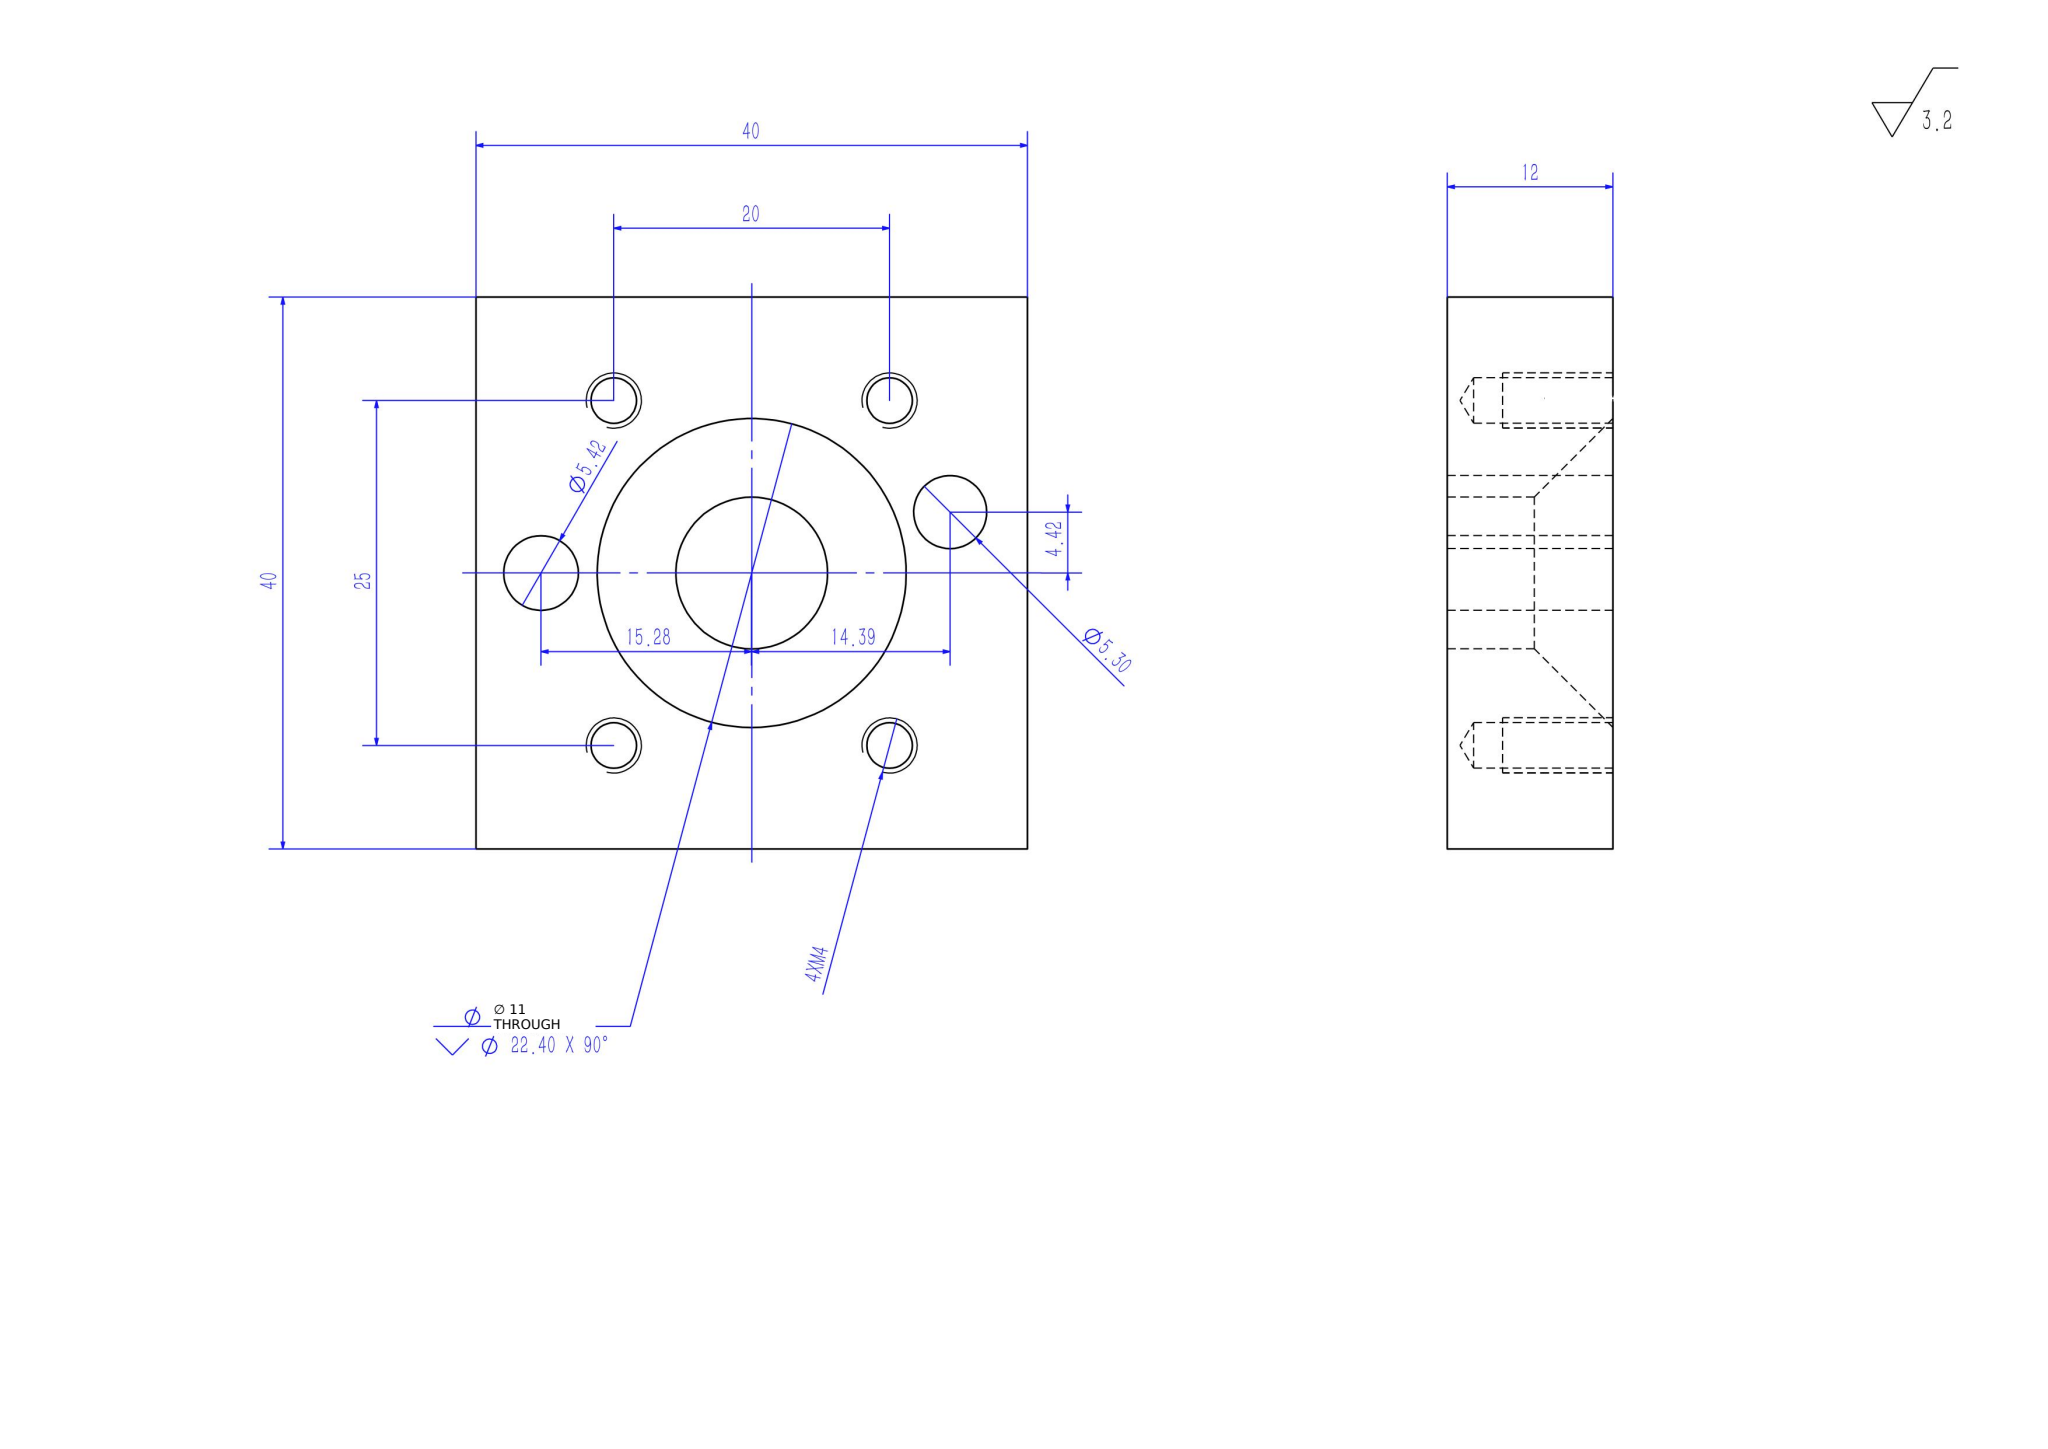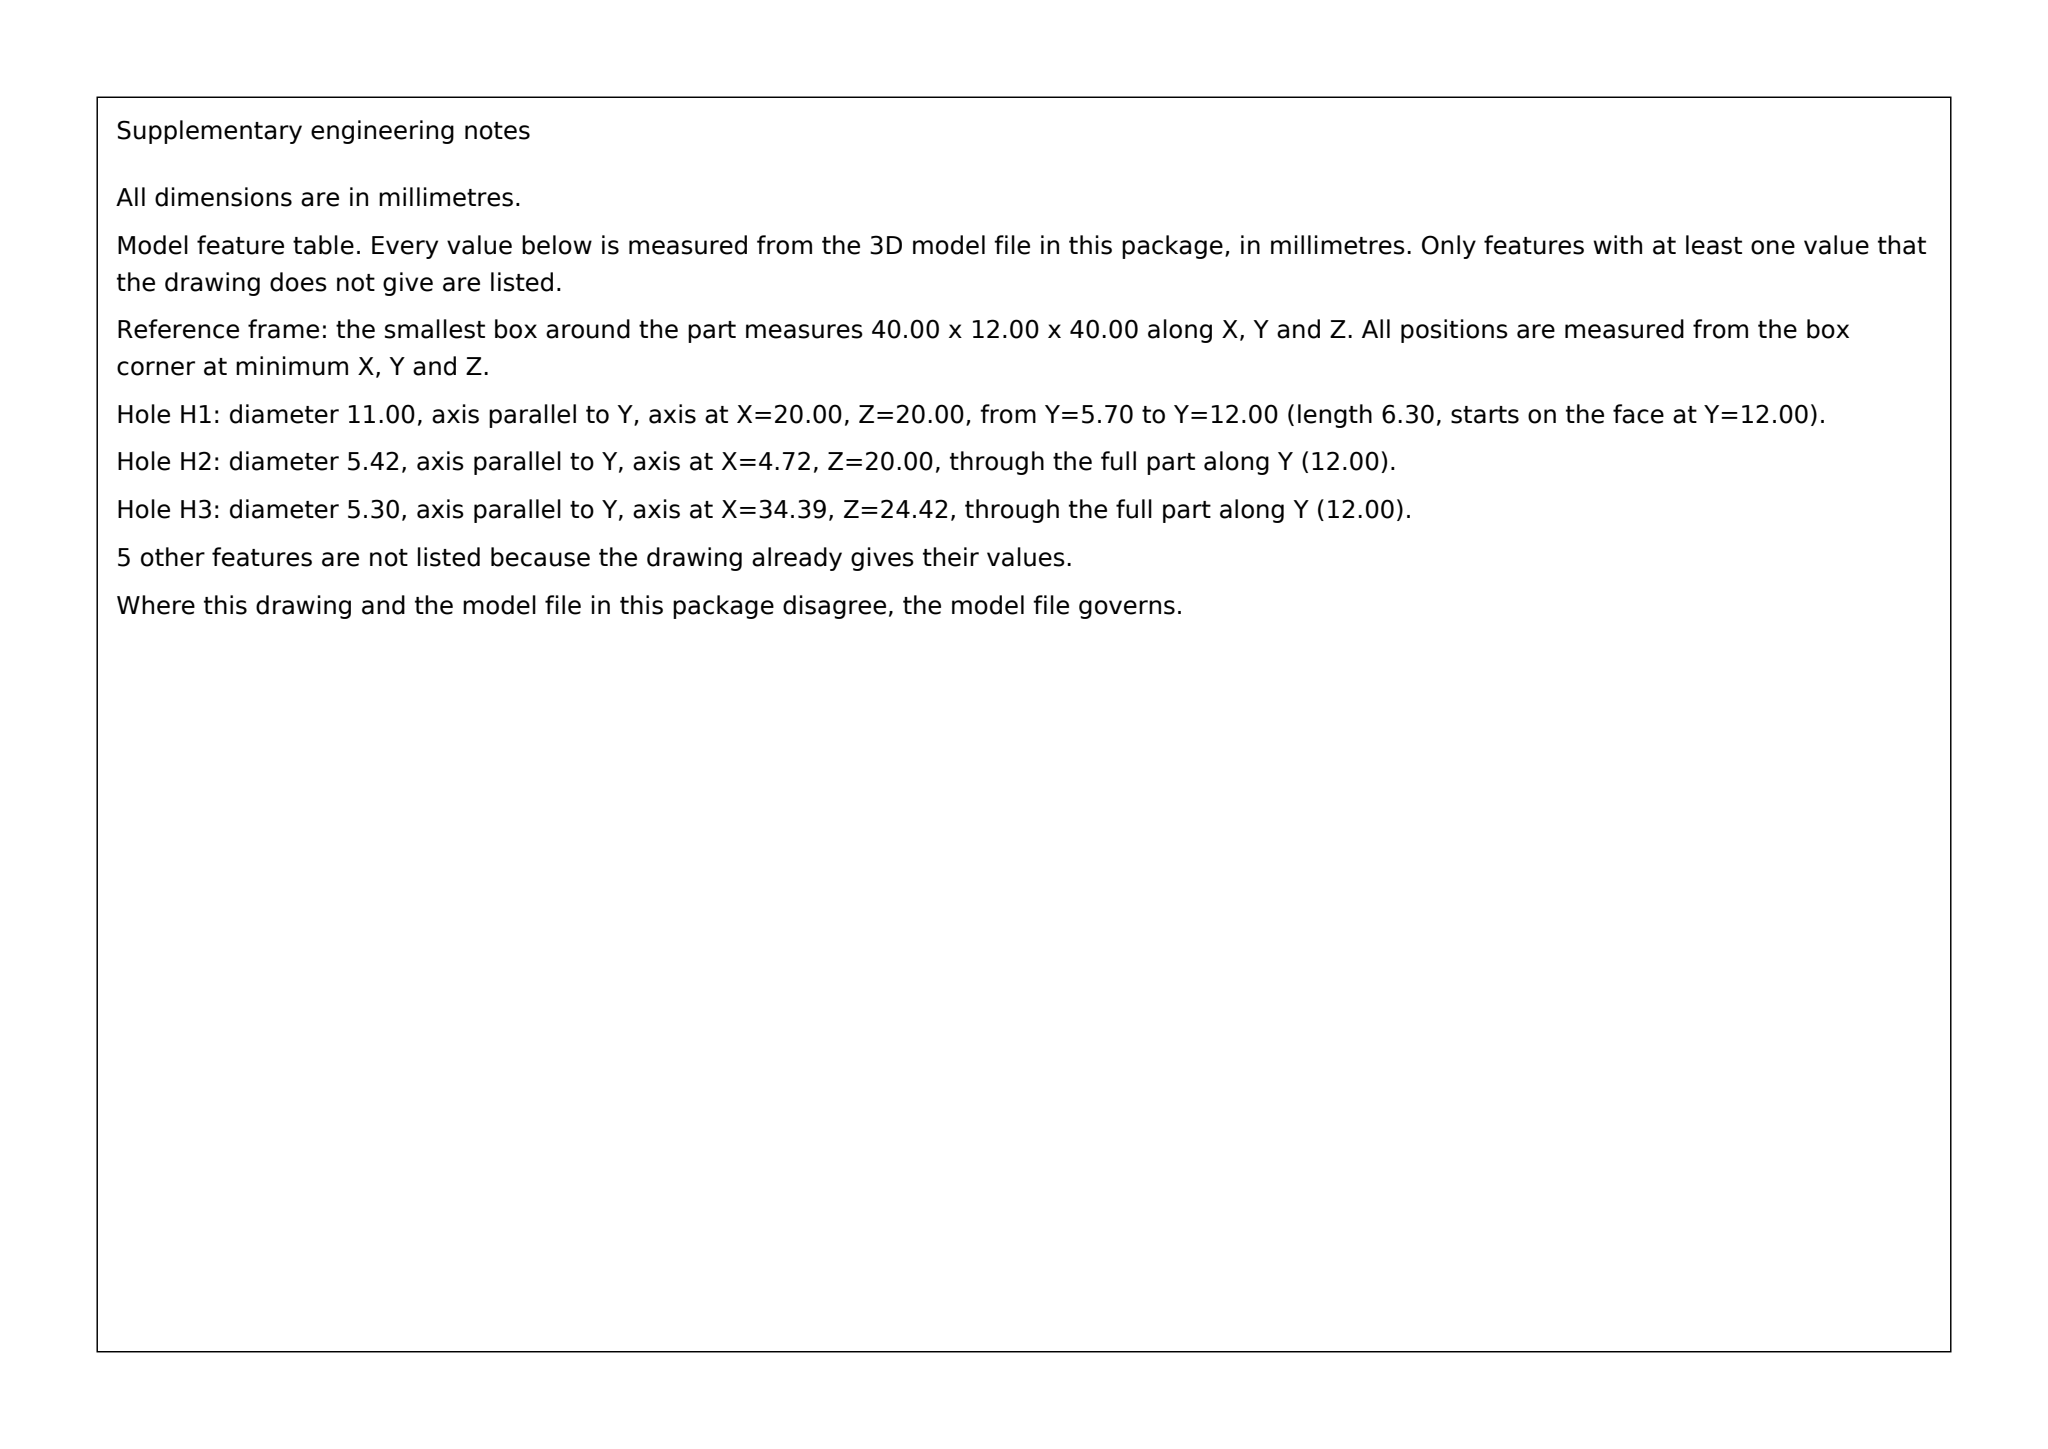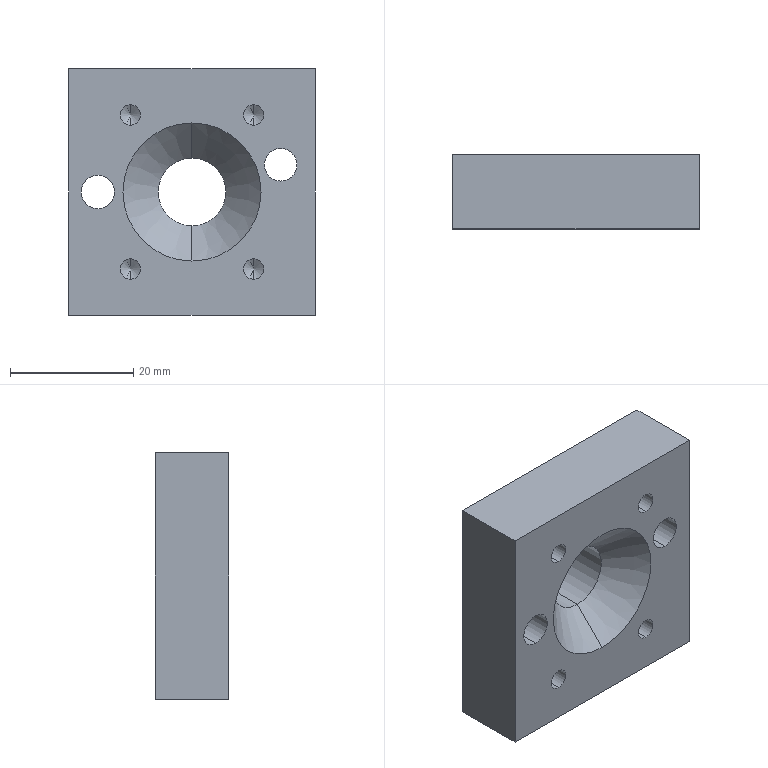Part | SolidWorks | mm | 1 solid | 30 faces | box 40 x 12 x 40 mm | volume 16406 mm3 | cylinder 14 | cone 10 | plane 6 | commonest cylinder face diameters 3.3 x8 5.298 x2 5.416 x2 11 x2
build123d program:
from build123d import *

# Parameters (mm, degrees)
SKETCH1_W                                        = 40
SKETCH1_H                                        = 40
BOSS_EXTRUDE1_DEPTH                              = 12
M10_HEX_SOCKET_HEAD_CAP_SCREW_CBORE1_D           = 11
M10_HEX_SOCKET_HEAD_CAP_SCREW_CBORE1_CSINK_D     = 22.4
M10_HEX_SOCKET_HEAD_CAP_SCREW_CBORE1_CSINK_ANGLE = 90
M4_TAPPED_HOLE1_D                                = 3.3
M4_TAPPED_HOLE1_DEPTH                            = 10.1
M4_TAPPED_HOLE1_TIP                              = 0.9914
SKETCH6_R                                        = 2.649
SKETCH6_R_2                                      = 2.708
CUT_EXTRUDE1_DEPTH                               = 80


with BuildPart() as part:
    # Sketch1 → Boss-Extrude1 (new body)
    with BuildSketch(Plane(origin=(0, 0, 0), x_dir=(1, 0, 0), z_dir=(0, 1, 0))):
        Rectangle(SKETCH1_W, SKETCH1_H)
    extrude(amount=BOSS_EXTRUDE1_DEPTH)

    # M10 Hex Socket Head Cap Screw CBORE1 (through all)
    with Locations(Plane(origin=(0, 0, 0), x_dir=(-1, 0, 0), z_dir=(0, -1, 0))):
        with Locations((0, 0)):
            CounterSinkHole(M10_HEX_SOCKET_HEAD_CAP_SCREW_CBORE1_D / 2, M10_HEX_SOCKET_HEAD_CAP_SCREW_CBORE1_CSINK_D / 2, counter_sink_angle=M10_HEX_SOCKET_HEAD_CAP_SCREW_CBORE1_CSINK_ANGLE)

    # M4 Tapped Hole1
    with Locations(Plane(origin=(0, 0, 0), x_dir=(-1, 0, 0), z_dir=(0, -1, 0))):
        with Locations((-10, 12.5), (10, 12.5), (-10, -12.5), (10, -12.5)):
            Hole(M4_TAPPED_HOLE1_D / 2, depth=M4_TAPPED_HOLE1_DEPTH)
            with Locations((0, 0, -(M4_TAPPED_HOLE1_DEPTH + M4_TAPPED_HOLE1_TIP / 2))):  # 118° drill point
                Cone(0, M4_TAPPED_HOLE1_D / 2, M4_TAPPED_HOLE1_TIP, mode=Mode.SUBTRACT)

    # Sketch6 → Cut-Extrude1 (cut)
    with BuildSketch(Plane(origin=(0, 0, 0), x_dir=(-1, 0, 0), z_dir=(0, -1, 0))):
        with Locations(Location((-14.39, -4.415, 0), (0, 0, 90))):
            Circle(SKETCH6_R)
        with Locations(Location((15.279, 0, 0), (0, 0, 90))):
            Circle(SKETCH6_R_2)
    extrude(amount=-CUT_EXTRUDE1_DEPTH, mode=Mode.SUBTRACT)


solid = part.part
STEP:
#1=CARTESIAN_POINT('',(14.39,12.,7.064));
#2=VERTEX_POINT('',#1);
#3=CARTESIAN_POINT('',(14.39,12.,1.766));
#4=VERTEX_POINT('',#3);
#5=CARTESIAN_POINT('',(14.39,12.,4.415));
#6=DIRECTION('',(0.,-1.,0.));
#7=DIRECTION('',(0.,0.,-1.));
#8=AXIS2_PLACEMENT_3D('',#5,#6,#7);
#9=CIRCLE('',#8,2.649);
#10=EDGE_CURVE('',#2,#4,#9,.T.);
#11=ORIENTED_EDGE('',*,*,#10,.F.);
#12=CARTESIAN_POINT('',(14.39,0.,7.064));
#13=VERTEX_POINT('',#12);
#14=CARTESIAN_POINT('',(14.39,80.,7.064));
#15=DIRECTION('',(0.,-1.,0.));
#16=VECTOR('',#15,1000.);
#17=LINE('',#14,#16);
#18=EDGE_CURVE('',#2,#13,#17,.T.);
#19=ORIENTED_EDGE('',*,*,#18,.T.);
#20=CARTESIAN_POINT('',(14.39,0.,1.766));
#21=VERTEX_POINT('',#20);
#22=CARTESIAN_POINT('',(14.39,0.,4.415));
#23=DIRECTION('',(0.,-1.,0.));
#24=DIRECTION('',(0.,0.,-1.));
#25=AXIS2_PLACEMENT_3D('',#22,#23,#24);
#26=CIRCLE('',#25,2.649);
#27=EDGE_CURVE('',#13,#21,#26,.T.);
#28=ORIENTED_EDGE('',*,*,#27,.T.);
#29=CARTESIAN_POINT('',(14.39,80.,1.766));
#30=DIRECTION('',(0.,-1.,0.));
#31=VECTOR('',#30,1000.);
#32=LINE('',#29,#31);
#33=EDGE_CURVE('',#4,#21,#32,.T.);
#34=ORIENTED_EDGE('',*,*,#33,.F.);
#35=EDGE_LOOP('',(#11,#19,#28,#34));
#36=FACE_OUTER_BOUND('',#35,.T.);
#37=CARTESIAN_POINT('',(14.39,80.,4.415));
#38=DIRECTION('',(0.,-1.,0.));
#39=DIRECTION('',(0.,0.,-1.));
#40=AXIS2_PLACEMENT_3D('',#37,#38,#39);
#41=CYLINDRICAL_SURFACE('',#40,2.649);
#42=ADVANCED_FACE('',(#36),#41,.F.);
#43=CARTESIAN_POINT('',(-15.279,12.,2.708));
#44=VERTEX_POINT('',#43);
#45=CARTESIAN_POINT('',(-15.279,12.,-2.708));
#46=VERTEX_POINT('',#45);
#47=CARTESIAN_POINT('',(-15.279,12.,0.));
#48=DIRECTION('',(0.,-1.,0.));
#49=DIRECTION('',(0.,0.,-1.));
#50=AXIS2_PLACEMENT_3D('',#47,#48,#49);
#51=CIRCLE('',#50,2.708);
#52=EDGE_CURVE('',#44,#46,#51,.T.);
#53=ORIENTED_EDGE('',*,*,#52,.F.);
#54=CARTESIAN_POINT('',(-15.279,0.,2.708));
#55=VERTEX_POINT('',#54);
#56=CARTESIAN_POINT('',(-15.279,80.,2.708));
#57=DIRECTION('',(0.,-1.,0.));
#58=VECTOR('',#57,1000.);
#59=LINE('',#56,#58);
#60=EDGE_CURVE('',#44,#55,#59,.T.);
#61=ORIENTED_EDGE('',*,*,#60,.T.);
#62=CARTESIAN_POINT('',(-15.279,0.,-2.708));
#63=VERTEX_POINT('',#62);
#64=CARTESIAN_POINT('',(-15.279,0.,0.));
#65=DIRECTION('',(0.,-1.,0.));
#66=DIRECTION('',(0.,0.,-1.));
#67=AXIS2_PLACEMENT_3D('',#64,#65,#66);
#68=CIRCLE('',#67,2.708);
#69=EDGE_CURVE('',#55,#63,#68,.T.);
#70=ORIENTED_EDGE('',*,*,#69,.T.);
#71=CARTESIAN_POINT('',(-15.279,80.,-2.708));
#72=DIRECTION('',(0.,-1.,0.));
#73=VECTOR('',#72,1000.);
#74=LINE('',#71,#73);
#75=EDGE_CURVE('',#46,#63,#74,.T.);
#76=ORIENTED_EDGE('',*,*,#75,.F.);
#77=EDGE_LOOP('',(#53,#61,#70,#76));
#78=FACE_OUTER_BOUND('',#77,.T.);
#79=CARTESIAN_POINT('',(-15.279,80.,0.));
#80=DIRECTION('',(0.,-1.,0.));
#81=DIRECTION('',(0.,0.,-1.));
#82=AXIS2_PLACEMENT_3D('',#79,#80,#81);
#83=CYLINDRICAL_SURFACE('',#82,2.708);
#84=ADVANCED_FACE('',(#78),#83,.F.);
#85=CARTESIAN_POINT('',(10.,10.1,-10.85));
#86=VERTEX_POINT('',#85);
#87=CARTESIAN_POINT('',(10.,10.1,-14.15));
#88=VERTEX_POINT('',#87);
#89=CARTESIAN_POINT('',(10.,10.1,-12.5));
#90=DIRECTION('',(0.,-1.,0.));
#91=DIRECTION('',(0.,0.,-1.));
#92=AXIS2_PLACEMENT_3D('',#89,#90,#91);
#93=CIRCLE('',#92,1.65);
#94=EDGE_CURVE('',#86,#88,#93,.T.);
#95=ORIENTED_EDGE('',*,*,#94,.F.);
#96=CARTESIAN_POINT('',(10.,-0.,-10.85));
#97=VERTEX_POINT('',#96);
#98=CARTESIAN_POINT('',(10.,0.,-10.85));
#99=DIRECTION('',(0.,-1.,0.));
#100=VECTOR('',#99,1000.);
#101=LINE('',#98,#100);
#102=EDGE_CURVE('',#86,#97,#101,.T.);
#103=ORIENTED_EDGE('',*,*,#102,.T.);
#104=CARTESIAN_POINT('',(10.,-0.,-14.15));
#105=VERTEX_POINT('',#104);
#106=CARTESIAN_POINT('',(10.,-0.,-12.5));
#107=DIRECTION('',(0.,-1.,0.));
#108=DIRECTION('',(0.,0.,-1.));
#109=AXIS2_PLACEMENT_3D('',#106,#107,#108);
#110=CIRCLE('',#109,1.65);
#111=EDGE_CURVE('',#97,#105,#110,.T.);
#112=ORIENTED_EDGE('',*,*,#111,.T.);
#113=CARTESIAN_POINT('',(10.,0.,-14.15));
#114=DIRECTION('',(0.,-1.,0.));
#115=VECTOR('',#114,1000.);
#116=LINE('',#113,#115);
#117=EDGE_CURVE('',#88,#105,#116,.T.);
#118=ORIENTED_EDGE('',*,*,#117,.F.);
#119=EDGE_LOOP('',(#95,#103,#112,#118));
#120=FACE_OUTER_BOUND('',#119,.T.);
#121=CARTESIAN_POINT('',(10.,0.,-12.5));
#122=DIRECTION('',(0.,-1.,0.));
#123=DIRECTION('',(0.,0.,-1.));
#124=AXIS2_PLACEMENT_3D('',#121,#122,#123);
#125=CYLINDRICAL_SURFACE('',#124,1.65);
#126=ADVANCED_FACE('',(#120),#125,.F.);
#127=CARTESIAN_POINT('',(10.,11.091,-12.5));
#128=VERTEX_POINT('',#127);
#129=CARTESIAN_POINT('',(10.,10.1,-14.15));
#130=DIRECTION('',(0.,-0.515,-0.8572));
#131=VECTOR('',#130,1000.);
#132=LINE('',#129,#131);
#133=EDGE_CURVE('',#128,#88,#132,.T.);
#134=ORIENTED_EDGE('',*,*,#133,.F.);
#135=CARTESIAN_POINT('',(10.,10.1,-10.85));
#136=DIRECTION('',(0.,-0.515,0.8572));
#137=VECTOR('',#136,1000.);
#138=LINE('',#135,#137);
#139=EDGE_CURVE('',#128,#86,#138,.T.);
#140=ORIENTED_EDGE('',*,*,#139,.T.);
#141=ORIENTED_EDGE('',*,*,#94,.T.);
#142=EDGE_LOOP('',(#134,#140,#141));
#143=FACE_OUTER_BOUND('',#142,.T.);
#144=CARTESIAN_POINT('',(10.,10.1,-12.5));
#145=DIRECTION('',(0.,-1.,0.));
#146=DIRECTION('',(0.,0.,-1.));
#147=AXIS2_PLACEMENT_3D('',#144,#145,#146);
#148=CONICAL_SURFACE('',#147,1.65,1.03);
#149=ADVANCED_FACE('',(#143),#148,.F.);
#150=CARTESIAN_POINT('',(-10.,10.1,-10.85));
#151=VERTEX_POINT('',#150);
#152=CARTESIAN_POINT('',(-10.,10.1,-14.15));
#153=VERTEX_POINT('',#152);
#154=CARTESIAN_POINT('',(-10.,10.1,-12.5));
#155=DIRECTION('',(0.,-1.,0.));
#156=DIRECTION('',(0.,0.,-1.));
#157=AXIS2_PLACEMENT_3D('',#154,#155,#156);
#158=CIRCLE('',#157,1.65);
#159=EDGE_CURVE('',#151,#153,#158,.T.);
#160=ORIENTED_EDGE('',*,*,#159,.F.);
#161=CARTESIAN_POINT('',(-10.,-0.,-10.85));
#162=VERTEX_POINT('',#161);
#163=CARTESIAN_POINT('',(-10.,0.,-10.85));
#164=DIRECTION('',(0.,-1.,0.));
#165=VECTOR('',#164,1000.);
#166=LINE('',#163,#165);
#167=EDGE_CURVE('',#151,#162,#166,.T.);
#168=ORIENTED_EDGE('',*,*,#167,.T.);
#169=CARTESIAN_POINT('',(-10.,-0.,-14.15));
#170=VERTEX_POINT('',#169);
#171=CARTESIAN_POINT('',(-10.,-0.,-12.5));
#172=DIRECTION('',(0.,-1.,0.));
#173=DIRECTION('',(0.,0.,-1.));
#174=AXIS2_PLACEMENT_3D('',#171,#172,#173);
#175=CIRCLE('',#174,1.65);
#176=EDGE_CURVE('',#162,#170,#175,.T.);
#177=ORIENTED_EDGE('',*,*,#176,.T.);
#178=CARTESIAN_POINT('',(-10.,0.,-14.15));
#179=DIRECTION('',(0.,-1.,0.));
#180=VECTOR('',#179,1000.);
#181=LINE('',#178,#180);
#182=EDGE_CURVE('',#153,#170,#181,.T.);
#183=ORIENTED_EDGE('',*,*,#182,.F.);
#184=EDGE_LOOP('',(#160,#168,#177,#183));
#185=FACE_OUTER_BOUND('',#184,.T.);
#186=CARTESIAN_POINT('',(-10.,0.,-12.5));
#187=DIRECTION('',(0.,-1.,0.));
#188=DIRECTION('',(0.,0.,-1.));
#189=AXIS2_PLACEMENT_3D('',#186,#187,#188);
#190=CYLINDRICAL_SURFACE('',#189,1.65);
#191=ADVANCED_FACE('',(#185),#190,.F.);
#192=CARTESIAN_POINT('',(-10.,11.091,-12.5));
#193=VERTEX_POINT('',#192);
#194=CARTESIAN_POINT('',(-10.,10.1,-14.15));
#195=DIRECTION('',(0.,-0.515,-0.8572));
#196=VECTOR('',#195,1000.);
#197=LINE('',#194,#196);
#198=EDGE_CURVE('',#193,#153,#197,.T.);
#199=ORIENTED_EDGE('',*,*,#198,.F.);
#200=CARTESIAN_POINT('',(-10.,10.1,-10.85));
#201=DIRECTION('',(0.,-0.515,0.8572));
#202=VECTOR('',#201,1000.);
#203=LINE('',#200,#202);
#204=EDGE_CURVE('',#193,#151,#203,.T.);
#205=ORIENTED_EDGE('',*,*,#204,.T.);
#206=ORIENTED_EDGE('',*,*,#159,.T.);
#207=EDGE_LOOP('',(#199,#205,#206));
#208=FACE_OUTER_BOUND('',#207,.T.);
#209=CARTESIAN_POINT('',(-10.,10.1,-12.5));
#210=DIRECTION('',(0.,-1.,0.));
#211=DIRECTION('',(0.,0.,-1.));
#212=AXIS2_PLACEMENT_3D('',#209,#210,#211);
#213=CONICAL_SURFACE('',#212,1.65,1.03);
#214=ADVANCED_FACE('',(#208),#213,.F.);
#215=CARTESIAN_POINT('',(10.,10.1,14.15));
#216=VERTEX_POINT('',#215);
#217=CARTESIAN_POINT('',(10.,10.1,10.85));
#218=VERTEX_POINT('',#217);
#219=CARTESIAN_POINT('',(10.,10.1,12.5));
#220=DIRECTION('',(0.,-1.,0.));
#221=DIRECTION('',(0.,0.,-1.));
#222=AXIS2_PLACEMENT_3D('',#219,#220,#221);
#223=CIRCLE('',#222,1.65);
#224=EDGE_CURVE('',#216,#218,#223,.T.);
#225=ORIENTED_EDGE('',*,*,#224,.F.);
#226=CARTESIAN_POINT('',(10.,-0.,14.15));
#227=VERTEX_POINT('',#226);
#228=CARTESIAN_POINT('',(10.,0.,14.15));
#229=DIRECTION('',(0.,-1.,0.));
#230=VECTOR('',#229,1000.);
#231=LINE('',#228,#230);
#232=EDGE_CURVE('',#216,#227,#231,.T.);
#233=ORIENTED_EDGE('',*,*,#232,.T.);
#234=CARTESIAN_POINT('',(10.,-0.,10.85));
#235=VERTEX_POINT('',#234);
#236=CARTESIAN_POINT('',(10.,-0.,12.5));
#237=DIRECTION('',(0.,-1.,0.));
#238=DIRECTION('',(0.,0.,-1.));
#239=AXIS2_PLACEMENT_3D('',#236,#237,#238);
#240=CIRCLE('',#239,1.65);
#241=EDGE_CURVE('',#227,#235,#240,.T.);
#242=ORIENTED_EDGE('',*,*,#241,.T.);
#243=CARTESIAN_POINT('',(10.,0.,10.85));
#244=DIRECTION('',(0.,-1.,0.));
#245=VECTOR('',#244,1000.);
#246=LINE('',#243,#245);
#247=EDGE_CURVE('',#218,#235,#246,.T.);
#248=ORIENTED_EDGE('',*,*,#247,.F.);
#249=EDGE_LOOP('',(#225,#233,#242,#248));
#250=FACE_OUTER_BOUND('',#249,.T.);
#251=CARTESIAN_POINT('',(10.,0.,12.5));
#252=DIRECTION('',(0.,-1.,0.));
#253=DIRECTION('',(0.,0.,-1.));
#254=AXIS2_PLACEMENT_3D('',#251,#252,#253);
#255=CYLINDRICAL_SURFACE('',#254,1.65);
#256=ADVANCED_FACE('',(#250),#255,.F.);
#257=CARTESIAN_POINT('',(10.,11.091,12.5));
#258=VERTEX_POINT('',#257);
#259=CARTESIAN_POINT('',(10.,10.1,10.85));
#260=DIRECTION('',(0.,-0.515,-0.8572));
#261=VECTOR('',#260,1000.);
#262=LINE('',#259,#261);
#263=EDGE_CURVE('',#258,#218,#262,.T.);
#264=ORIENTED_EDGE('',*,*,#263,.F.);
#265=CARTESIAN_POINT('',(10.,10.1,14.15));
#266=DIRECTION('',(0.,-0.515,0.8572));
#267=VECTOR('',#266,1000.);
#268=LINE('',#265,#267);
#269=EDGE_CURVE('',#258,#216,#268,.T.);
#270=ORIENTED_EDGE('',*,*,#269,.T.);
#271=ORIENTED_EDGE('',*,*,#224,.T.);
#272=EDGE_LOOP('',(#264,#270,#271));
#273=FACE_OUTER_BOUND('',#272,.T.);
#274=CARTESIAN_POINT('',(10.,10.1,12.5));
#275=DIRECTION('',(0.,-1.,0.));
#276=DIRECTION('',(0.,0.,-1.));
#277=AXIS2_PLACEMENT_3D('',#274,#275,#276);
#278=CONICAL_SURFACE('',#277,1.65,1.03);
#279=ADVANCED_FACE('',(#273),#278,.F.);
#280=CARTESIAN_POINT('',(-10.,10.1,14.15));
#281=VERTEX_POINT('',#280);
#282=CARTESIAN_POINT('',(-10.,10.1,10.85));
#283=VERTEX_POINT('',#282);
#284=CARTESIAN_POINT('',(-10.,10.1,12.5));
#285=DIRECTION('',(0.,-1.,0.));
#286=DIRECTION('',(0.,0.,-1.));
#287=AXIS2_PLACEMENT_3D('',#284,#285,#286);
#288=CIRCLE('',#287,1.65);
#289=EDGE_CURVE('',#281,#283,#288,.T.);
#290=ORIENTED_EDGE('',*,*,#289,.F.);
#291=CARTESIAN_POINT('',(-10.,-0.,14.15));
#292=VERTEX_POINT('',#291);
#293=CARTESIAN_POINT('',(-10.,0.,14.15));
#294=DIRECTION('',(0.,-1.,0.));
#295=VECTOR('',#294,1000.);
#296=LINE('',#293,#295);
#297=EDGE_CURVE('',#281,#292,#296,.T.);
#298=ORIENTED_EDGE('',*,*,#297,.T.);
#299=CARTESIAN_POINT('',(-10.,-0.,10.85));
#300=VERTEX_POINT('',#299);
#301=CARTESIAN_POINT('',(-10.,-0.,12.5));
#302=DIRECTION('',(0.,-1.,0.));
#303=DIRECTION('',(0.,0.,-1.));
#304=AXIS2_PLACEMENT_3D('',#301,#302,#303);
#305=CIRCLE('',#304,1.65);
#306=EDGE_CURVE('',#292,#300,#305,.T.);
#307=ORIENTED_EDGE('',*,*,#306,.T.);
#308=CARTESIAN_POINT('',(-10.,0.,10.85));
#309=DIRECTION('',(0.,-1.,0.));
#310=VECTOR('',#309,1000.);
#311=LINE('',#308,#310);
#312=EDGE_CURVE('',#283,#300,#311,.T.);
#313=ORIENTED_EDGE('',*,*,#312,.F.);
#314=EDGE_LOOP('',(#290,#298,#307,#313));
#315=FACE_OUTER_BOUND('',#314,.T.);
#316=CARTESIAN_POINT('',(-10.,0.,12.5));
#317=DIRECTION('',(0.,-1.,0.));
#318=DIRECTION('',(0.,0.,-1.));
#319=AXIS2_PLACEMENT_3D('',#316,#317,#318);
#320=CYLINDRICAL_SURFACE('',#319,1.65);
#321=ADVANCED_FACE('',(#315),#320,.F.);
#322=CARTESIAN_POINT('',(-10.,11.091,12.5));
#323=VERTEX_POINT('',#322);
#324=CARTESIAN_POINT('',(-10.,10.1,10.85));
#325=DIRECTION('',(0.,-0.515,-0.8572));
#326=VECTOR('',#325,1000.);
#327=LINE('',#324,#326);
#328=EDGE_CURVE('',#323,#283,#327,.T.);
#329=ORIENTED_EDGE('',*,*,#328,.F.);
#330=CARTESIAN_POINT('',(-10.,10.1,14.15));
#331=DIRECTION('',(0.,-0.515,0.8572));
#332=VECTOR('',#331,1000.);
#333=LINE('',#330,#332);
#334=EDGE_CURVE('',#323,#281,#333,.T.);
#335=ORIENTED_EDGE('',*,*,#334,.T.);
#336=ORIENTED_EDGE('',*,*,#289,.T.);
#337=EDGE_LOOP('',(#329,#335,#336));
#338=FACE_OUTER_BOUND('',#337,.T.);
#339=CARTESIAN_POINT('',(-10.,10.1,12.5));
#340=DIRECTION('',(0.,-1.,0.));
#341=DIRECTION('',(0.,0.,-1.));
#342=AXIS2_PLACEMENT_3D('',#339,#340,#341);
#343=CONICAL_SURFACE('',#342,1.65,1.03);
#344=ADVANCED_FACE('',(#338),#343,.F.);
#345=CARTESIAN_POINT('',(-0.,5.7,5.5));
#346=VERTEX_POINT('',#345);
#347=CARTESIAN_POINT('',(-0.,5.7,-5.5));
#348=VERTEX_POINT('',#347);
#349=CARTESIAN_POINT('',(-0.,5.7,-0.));
#350=DIRECTION('',(0.,-1.,0.));
#351=DIRECTION('',(0.,0.,-1.));
#352=AXIS2_PLACEMENT_3D('',#349,#350,#351);
#353=CIRCLE('',#352,5.5);
#354=EDGE_CURVE('',#346,#348,#353,.T.);
#355=ORIENTED_EDGE('',*,*,#354,.F.);
#356=CARTESIAN_POINT('',(-0.,-0.,11.2));
#357=VERTEX_POINT('',#356);
#358=CARTESIAN_POINT('',(-0.,-0.,11.2));
#359=DIRECTION('',(0.,-0.7071,0.7071));
#360=VECTOR('',#359,1000.);
#361=LINE('',#358,#360);
#362=EDGE_CURVE('',#346,#357,#361,.T.);
#363=ORIENTED_EDGE('',*,*,#362,.T.);
#364=CARTESIAN_POINT('',(-0.,-0.,-11.2));
#365=VERTEX_POINT('',#364);
#366=CARTESIAN_POINT('',(-0.,-0.,-0.));
#367=DIRECTION('',(0.,-1.,0.));
#368=DIRECTION('',(0.,0.,-1.));
#369=AXIS2_PLACEMENT_3D('',#366,#367,#368);
#370=CIRCLE('',#369,11.2);
#371=EDGE_CURVE('',#357,#365,#370,.T.);
#372=ORIENTED_EDGE('',*,*,#371,.T.);
#373=CARTESIAN_POINT('',(-0.,-0.,-11.2));
#374=DIRECTION('',(0.,-0.7071,-0.7071));
#375=VECTOR('',#374,1000.);
#376=LINE('',#373,#375);
#377=EDGE_CURVE('',#348,#365,#376,.T.);
#378=ORIENTED_EDGE('',*,*,#377,.F.);
#379=EDGE_LOOP('',(#355,#363,#372,#378));
#380=FACE_OUTER_BOUND('',#379,.T.);
#381=CARTESIAN_POINT('',(-0.,-0.,-0.));
#382=DIRECTION('',(0.,-1.,0.));
#383=DIRECTION('',(0.,0.,-1.));
#384=AXIS2_PLACEMENT_3D('',#381,#382,#383);
#385=CONICAL_SURFACE('',#384,11.2,0.7854);
#386=ADVANCED_FACE('',(#380),#385,.F.);
#387=CARTESIAN_POINT('',(-0.,12.,5.5));
#388=VERTEX_POINT('',#387);
#389=CARTESIAN_POINT('',(-0.,12.,-5.5));
#390=VERTEX_POINT('',#389);
#391=CARTESIAN_POINT('',(-0.,12.,-0.));
#392=DIRECTION('',(0.,-1.,0.));
#393=DIRECTION('',(0.,0.,-1.));
#394=AXIS2_PLACEMENT_3D('',#391,#392,#393);
#395=CIRCLE('',#394,5.5);
#396=EDGE_CURVE('',#388,#390,#395,.T.);
#397=ORIENTED_EDGE('',*,*,#396,.F.);
#398=CARTESIAN_POINT('',(-0.,0.,5.5));
#399=DIRECTION('',(0.,-1.,0.));
#400=VECTOR('',#399,1000.);
#401=LINE('',#398,#400);
#402=EDGE_CURVE('',#388,#346,#401,.T.);
#403=ORIENTED_EDGE('',*,*,#402,.T.);
#404=ORIENTED_EDGE('',*,*,#354,.T.);
#405=CARTESIAN_POINT('',(-0.,0.,-5.5));
#406=DIRECTION('',(0.,-1.,0.));
#407=VECTOR('',#406,1000.);
#408=LINE('',#405,#407);
#409=EDGE_CURVE('',#390,#348,#408,.T.);
#410=ORIENTED_EDGE('',*,*,#409,.F.);
#411=EDGE_LOOP('',(#397,#403,#404,#410));
#412=FACE_OUTER_BOUND('',#411,.T.);
#413=CARTESIAN_POINT('',(-0.,0.,-0.));
#414=DIRECTION('',(0.,-1.,0.));
#415=DIRECTION('',(0.,0.,-1.));
#416=AXIS2_PLACEMENT_3D('',#413,#414,#415);
#417=CYLINDRICAL_SURFACE('',#416,5.5);
#418=ADVANCED_FACE('',(#412),#417,.F.);
#419=CARTESIAN_POINT('',(20.,0.,20.));
#420=VERTEX_POINT('',#419);
#421=CARTESIAN_POINT('',(20.,0.,-20.));
#422=VERTEX_POINT('',#421);
#423=CARTESIAN_POINT('',(20.,0.,20.));
#424=DIRECTION('',(0.,0.,-1.));
#425=VECTOR('',#424,1000.);
#426=LINE('',#423,#425);
#427=EDGE_CURVE('',#420,#422,#426,.T.);
#428=ORIENTED_EDGE('',*,*,#427,.T.);
#429=CARTESIAN_POINT('',(20.,12.,-20.));
#430=VERTEX_POINT('',#429);
#431=CARTESIAN_POINT('',(20.,12.,-20.));
#432=DIRECTION('',(0.,-1.,0.));
#433=VECTOR('',#432,1000.);
#434=LINE('',#431,#433);
#435=EDGE_CURVE('',#430,#422,#434,.T.);
#436=ORIENTED_EDGE('',*,*,#435,.F.);
#437=CARTESIAN_POINT('',(20.,12.,20.));
#438=VERTEX_POINT('',#437);
#439=CARTESIAN_POINT('',(20.,12.,20.));
#440=DIRECTION('',(0.,0.,-1.));
#441=VECTOR('',#440,1000.);
#442=LINE('',#439,#441);
#443=EDGE_CURVE('',#438,#430,#442,.T.);
#444=ORIENTED_EDGE('',*,*,#443,.F.);
#445=CARTESIAN_POINT('',(20.,12.,20.));
#446=DIRECTION('',(0.,-1.,0.));
#447=VECTOR('',#446,1000.);
#448=LINE('',#445,#447);
#449=EDGE_CURVE('',#438,#420,#448,.T.);
#450=ORIENTED_EDGE('',*,*,#449,.T.);
#451=EDGE_LOOP('',(#428,#436,#444,#450));
#452=FACE_OUTER_BOUND('',#451,.T.);
#453=CARTESIAN_POINT('',(20.,12.,20.));
#454=DIRECTION('',(-1.,0.,0.));
#455=DIRECTION('',(0.,0.,1.));
#456=AXIS2_PLACEMENT_3D('',#453,#454,#455);
#457=PLANE('',#456);
#458=ADVANCED_FACE('',(#452),#457,.F.);
#459=CARTESIAN_POINT('',(-20.,0.,-20.));
#460=VERTEX_POINT('',#459);
#461=CARTESIAN_POINT('',(-20.,0.,-20.));
#462=DIRECTION('',(-1.,0.,0.));
#463=VECTOR('',#462,1000.);
#464=LINE('',#461,#463);
#465=EDGE_CURVE('',#422,#460,#464,.T.);
#466=ORIENTED_EDGE('',*,*,#465,.T.);
#467=CARTESIAN_POINT('',(-20.,12.,-20.));
#468=VERTEX_POINT('',#467);
#469=CARTESIAN_POINT('',(-20.,12.,-20.));
#470=DIRECTION('',(0.,-1.,0.));
#471=VECTOR('',#470,1000.);
#472=LINE('',#469,#471);
#473=EDGE_CURVE('',#468,#460,#472,.T.);
#474=ORIENTED_EDGE('',*,*,#473,.F.);
#475=CARTESIAN_POINT('',(-20.,12.,-20.));
#476=DIRECTION('',(-1.,0.,0.));
#477=VECTOR('',#476,1000.);
#478=LINE('',#475,#477);
#479=EDGE_CURVE('',#430,#468,#478,.T.);
#480=ORIENTED_EDGE('',*,*,#479,.F.);
#481=ORIENTED_EDGE('',*,*,#435,.T.);
#482=EDGE_LOOP('',(#466,#474,#480,#481));
#483=FACE_OUTER_BOUND('',#482,.T.);
#484=CARTESIAN_POINT('',(-20.,12.,-20.));
#485=DIRECTION('',(0.,0.,1.));
#486=DIRECTION('',(1.,0.,0.));
#487=AXIS2_PLACEMENT_3D('',#484,#485,#486);
#488=PLANE('',#487);
#489=ADVANCED_FACE('',(#483),#488,.F.);
#490=CARTESIAN_POINT('',(-20.,0.,20.));
#491=VERTEX_POINT('',#490);
#492=CARTESIAN_POINT('',(-20.,0.,20.));
#493=DIRECTION('',(0.,0.,1.));
#494=VECTOR('',#493,1000.);
#495=LINE('',#492,#494);
#496=EDGE_CURVE('',#460,#491,#495,.T.);
#497=ORIENTED_EDGE('',*,*,#496,.T.);
#498=CARTESIAN_POINT('',(-20.,12.,20.));
#499=VERTEX_POINT('',#498);
#500=CARTESIAN_POINT('',(-20.,12.,20.));
#501=DIRECTION('',(0.,-1.,0.));
#502=VECTOR('',#501,1000.);
#503=LINE('',#500,#502);
#504=EDGE_CURVE('',#499,#491,#503,.T.);
#505=ORIENTED_EDGE('',*,*,#504,.F.);
#506=CARTESIAN_POINT('',(-20.,12.,20.));
#507=DIRECTION('',(0.,0.,1.));
#508=VECTOR('',#507,1000.);
#509=LINE('',#506,#508);
#510=EDGE_CURVE('',#468,#499,#509,.T.);
#511=ORIENTED_EDGE('',*,*,#510,.F.);
#512=ORIENTED_EDGE('',*,*,#473,.T.);
#513=EDGE_LOOP('',(#497,#505,#511,#512));
#514=FACE_OUTER_BOUND('',#513,.T.);
#515=CARTESIAN_POINT('',(-20.,12.,20.));
#516=DIRECTION('',(1.,0.,0.));
#517=DIRECTION('',(0.,0.,-1.));
#518=AXIS2_PLACEMENT_3D('',#515,#516,#517);
#519=PLANE('',#518);
#520=ADVANCED_FACE('',(#514),#519,.F.);
#521=CARTESIAN_POINT('',(-20.,0.,20.));
#522=DIRECTION('',(1.,0.,0.));
#523=VECTOR('',#522,1000.);
#524=LINE('',#521,#523);
#525=EDGE_CURVE('',#491,#420,#524,.T.);
#526=ORIENTED_EDGE('',*,*,#525,.T.);
#527=ORIENTED_EDGE('',*,*,#449,.F.);
#528=CARTESIAN_POINT('',(-20.,12.,20.));
#529=DIRECTION('',(1.,0.,0.));
#530=VECTOR('',#529,1000.);
#531=LINE('',#528,#530);
#532=EDGE_CURVE('',#499,#438,#531,.T.);
#533=ORIENTED_EDGE('',*,*,#532,.F.);
#534=ORIENTED_EDGE('',*,*,#504,.T.);
#535=EDGE_LOOP('',(#526,#527,#533,#534));
#536=FACE_OUTER_BOUND('',#535,.T.);
#537=CARTESIAN_POINT('',(-20.,12.,20.));
#538=DIRECTION('',(0.,0.,-1.));
#539=DIRECTION('',(-1.,0.,0.));
#540=AXIS2_PLACEMENT_3D('',#537,#538,#539);
#541=PLANE('',#540);
#542=ADVANCED_FACE('',(#536),#541,.F.);
#543=CARTESIAN_POINT('',(14.39,12.,4.415));
#544=DIRECTION('',(0.,-1.,0.));
#545=DIRECTION('',(0.,0.,-1.));
#546=AXIS2_PLACEMENT_3D('',#543,#544,#545);
#547=CIRCLE('',#546,2.649);
#548=EDGE_CURVE('',#4,#2,#547,.T.);
#549=ORIENTED_EDGE('',*,*,#548,.T.);
#550=ORIENTED_EDGE('',*,*,#10,.T.);
#551=EDGE_LOOP('',(#549,#550));
#552=FACE_BOUND('',#551,.T.);
#553=CARTESIAN_POINT('',(-15.279,12.,0.));
#554=DIRECTION('',(0.,-1.,0.));
#555=DIRECTION('',(0.,0.,-1.));
#556=AXIS2_PLACEMENT_3D('',#553,#554,#555);
#557=CIRCLE('',#556,2.708);
#558=EDGE_CURVE('',#46,#44,#557,.T.);
#559=ORIENTED_EDGE('',*,*,#558,.T.);
#560=ORIENTED_EDGE('',*,*,#52,.T.);
#561=EDGE_LOOP('',(#559,#560));
#562=FACE_BOUND('',#561,.T.);
#563=CARTESIAN_POINT('',(-0.,12.,-0.));
#564=DIRECTION('',(0.,-1.,0.));
#565=DIRECTION('',(0.,0.,-1.));
#566=AXIS2_PLACEMENT_3D('',#563,#564,#565);
#567=CIRCLE('',#566,5.5);
#568=EDGE_CURVE('',#390,#388,#567,.T.);
#569=ORIENTED_EDGE('',*,*,#568,.T.);
#570=ORIENTED_EDGE('',*,*,#396,.T.);
#571=EDGE_LOOP('',(#569,#570));
#572=FACE_BOUND('',#571,.T.);
#573=ORIENTED_EDGE('',*,*,#443,.T.);
#574=ORIENTED_EDGE('',*,*,#479,.T.);
#575=ORIENTED_EDGE('',*,*,#510,.T.);
#576=ORIENTED_EDGE('',*,*,#532,.T.);
#577=EDGE_LOOP('',(#573,#574,#575,#576));
#578=FACE_OUTER_BOUND('',#577,.T.);
#579=CARTESIAN_POINT('',(0.,12.,0.));
#580=DIRECTION('',(0.,-1.,0.));
#581=DIRECTION('',(0.,0.,-1.));
#582=AXIS2_PLACEMENT_3D('',#579,#580,#581);
#583=PLANE('',#582);
#584=ADVANCED_FACE('',(#552,#562,#572,#578),#583,.F.);
#585=CARTESIAN_POINT('',(14.39,0.,4.415));
#586=DIRECTION('',(0.,-1.,0.));
#587=DIRECTION('',(0.,0.,-1.));
#588=AXIS2_PLACEMENT_3D('',#585,#586,#587);
#589=CIRCLE('',#588,2.649);
#590=EDGE_CURVE('',#21,#13,#589,.T.);
#591=ORIENTED_EDGE('',*,*,#590,.F.);
#592=ORIENTED_EDGE('',*,*,#27,.F.);
#593=EDGE_LOOP('',(#591,#592));
#594=FACE_BOUND('',#593,.T.);
#595=CARTESIAN_POINT('',(-15.279,0.,0.));
#596=DIRECTION('',(0.,-1.,0.));
#597=DIRECTION('',(0.,0.,-1.));
#598=AXIS2_PLACEMENT_3D('',#595,#596,#597);
#599=CIRCLE('',#598,2.708);
#600=EDGE_CURVE('',#63,#55,#599,.T.);
#601=ORIENTED_EDGE('',*,*,#600,.F.);
#602=ORIENTED_EDGE('',*,*,#69,.F.);
#603=EDGE_LOOP('',(#601,#602));
#604=FACE_BOUND('',#603,.T.);
#605=CARTESIAN_POINT('',(10.,-0.,-12.5));
#606=DIRECTION('',(0.,-1.,0.));
#607=DIRECTION('',(0.,0.,-1.));
#608=AXIS2_PLACEMENT_3D('',#605,#606,#607);
#609=CIRCLE('',#608,1.65);
#610=EDGE_CURVE('',#105,#97,#609,.T.);
#611=ORIENTED_EDGE('',*,*,#610,.F.);
#612=ORIENTED_EDGE('',*,*,#111,.F.);
#613=EDGE_LOOP('',(#611,#612));
#614=FACE_BOUND('',#613,.T.);
#615=CARTESIAN_POINT('',(-10.,-0.,-12.5));
#616=DIRECTION('',(0.,-1.,0.));
#617=DIRECTION('',(0.,0.,-1.));
#618=AXIS2_PLACEMENT_3D('',#615,#616,#617);
#619=CIRCLE('',#618,1.65);
#620=EDGE_CURVE('',#170,#162,#619,.T.);
#621=ORIENTED_EDGE('',*,*,#620,.F.);
#622=ORIENTED_EDGE('',*,*,#176,.F.);
#623=EDGE_LOOP('',(#621,#622));
#624=FACE_BOUND('',#623,.T.);
#625=CARTESIAN_POINT('',(10.,-0.,12.5));
#626=DIRECTION('',(0.,-1.,0.));
#627=DIRECTION('',(0.,0.,-1.));
#628=AXIS2_PLACEMENT_3D('',#625,#626,#627);
#629=CIRCLE('',#628,1.65);
#630=EDGE_CURVE('',#235,#227,#629,.T.);
#631=ORIENTED_EDGE('',*,*,#630,.F.);
#632=ORIENTED_EDGE('',*,*,#241,.F.);
#633=EDGE_LOOP('',(#631,#632));
#634=FACE_BOUND('',#633,.T.);
#635=CARTESIAN_POINT('',(-10.,-0.,12.5));
#636=DIRECTION('',(0.,-1.,0.));
#637=DIRECTION('',(0.,0.,-1.));
#638=AXIS2_PLACEMENT_3D('',#635,#636,#637);
#639=CIRCLE('',#638,1.65);
#640=EDGE_CURVE('',#300,#292,#639,.T.);
#641=ORIENTED_EDGE('',*,*,#640,.F.);
#642=ORIENTED_EDGE('',*,*,#306,.F.);
#643=EDGE_LOOP('',(#641,#642));
#644=FACE_BOUND('',#643,.T.);
#645=CARTESIAN_POINT('',(-0.,-0.,-0.));
#646=DIRECTION('',(0.,-1.,0.));
#647=DIRECTION('',(0.,0.,-1.));
#648=AXIS2_PLACEMENT_3D('',#645,#646,#647);
#649=CIRCLE('',#648,11.2);
#650=EDGE_CURVE('',#365,#357,#649,.T.);
#651=ORIENTED_EDGE('',*,*,#650,.F.);
#652=ORIENTED_EDGE('',*,*,#371,.F.);
#653=EDGE_LOOP('',(#651,#652));
#654=FACE_BOUND('',#653,.T.);
#655=ORIENTED_EDGE('',*,*,#427,.F.);
#656=ORIENTED_EDGE('',*,*,#525,.F.);
#657=ORIENTED_EDGE('',*,*,#496,.F.);
#658=ORIENTED_EDGE('',*,*,#465,.F.);
#659=EDGE_LOOP('',(#655,#656,#657,#658));
#660=FACE_OUTER_BOUND('',#659,.T.);
#661=CARTESIAN_POINT('',(0.,0.,0.));
#662=DIRECTION('',(0.,-1.,0.));
#663=DIRECTION('',(0.,0.,-1.));
#664=AXIS2_PLACEMENT_3D('',#661,#662,#663);
#665=PLANE('',#664);
#666=ADVANCED_FACE('',(#594,#604,#614,#624,#634,#644,#654,#660),#665,.T.);
#667=ORIENTED_EDGE('',*,*,#402,.F.);
#668=ORIENTED_EDGE('',*,*,#568,.F.);
#669=ORIENTED_EDGE('',*,*,#409,.T.);
#670=CARTESIAN_POINT('',(-0.,5.7,-0.));
#671=DIRECTION('',(0.,-1.,0.));
#672=DIRECTION('',(0.,0.,-1.));
#673=AXIS2_PLACEMENT_3D('',#670,#671,#672);
#674=CIRCLE('',#673,5.5);
#675=EDGE_CURVE('',#348,#346,#674,.T.);
#676=ORIENTED_EDGE('',*,*,#675,.T.);
#677=EDGE_LOOP('',(#667,#668,#669,#676));
#678=FACE_OUTER_BOUND('',#677,.T.);
#679=CARTESIAN_POINT('',(-0.,0.,-0.));
#680=DIRECTION('',(0.,-1.,0.));
#681=DIRECTION('',(0.,0.,-1.));
#682=AXIS2_PLACEMENT_3D('',#679,#680,#681);
#683=CYLINDRICAL_SURFACE('',#682,5.5);
#684=ADVANCED_FACE('',(#678),#683,.F.);
#685=ORIENTED_EDGE('',*,*,#362,.F.);
#686=ORIENTED_EDGE('',*,*,#675,.F.);
#687=ORIENTED_EDGE('',*,*,#377,.T.);
#688=ORIENTED_EDGE('',*,*,#650,.T.);
#689=EDGE_LOOP('',(#685,#686,#687,#688));
#690=FACE_OUTER_BOUND('',#689,.T.);
#691=CARTESIAN_POINT('',(-0.,-0.,-0.));
#692=DIRECTION('',(0.,-1.,0.));
#693=DIRECTION('',(0.,0.,-1.));
#694=AXIS2_PLACEMENT_3D('',#691,#692,#693);
#695=CONICAL_SURFACE('',#694,11.2,0.7854);
#696=ADVANCED_FACE('',(#690),#695,.F.);
#697=ORIENTED_EDGE('',*,*,#334,.F.);
#698=ORIENTED_EDGE('',*,*,#328,.T.);
#699=CARTESIAN_POINT('',(-10.,10.1,12.5));
#700=DIRECTION('',(0.,-1.,0.));
#701=DIRECTION('',(0.,0.,-1.));
#702=AXIS2_PLACEMENT_3D('',#699,#700,#701);
#703=CIRCLE('',#702,1.65);
#704=EDGE_CURVE('',#283,#281,#703,.T.);
#705=ORIENTED_EDGE('',*,*,#704,.T.);
#706=EDGE_LOOP('',(#697,#698,#705));
#707=FACE_OUTER_BOUND('',#706,.T.);
#708=CARTESIAN_POINT('',(-10.,10.1,12.5));
#709=DIRECTION('',(0.,-1.,0.));
#710=DIRECTION('',(0.,0.,-1.));
#711=AXIS2_PLACEMENT_3D('',#708,#709,#710);
#712=CONICAL_SURFACE('',#711,1.65,1.03);
#713=ADVANCED_FACE('',(#707),#712,.F.);
#714=ORIENTED_EDGE('',*,*,#297,.F.);
#715=ORIENTED_EDGE('',*,*,#704,.F.);
#716=ORIENTED_EDGE('',*,*,#312,.T.);
#717=ORIENTED_EDGE('',*,*,#640,.T.);
#718=EDGE_LOOP('',(#714,#715,#716,#717));
#719=FACE_OUTER_BOUND('',#718,.T.);
#720=CARTESIAN_POINT('',(-10.,0.,12.5));
#721=DIRECTION('',(0.,-1.,0.));
#722=DIRECTION('',(0.,0.,-1.));
#723=AXIS2_PLACEMENT_3D('',#720,#721,#722);
#724=CYLINDRICAL_SURFACE('',#723,1.65);
#725=ADVANCED_FACE('',(#719),#724,.F.);
#726=ORIENTED_EDGE('',*,*,#269,.F.);
#727=ORIENTED_EDGE('',*,*,#263,.T.);
#728=CARTESIAN_POINT('',(10.,10.1,12.5));
#729=DIRECTION('',(0.,-1.,0.));
#730=DIRECTION('',(0.,0.,-1.));
#731=AXIS2_PLACEMENT_3D('',#728,#729,#730);
#732=CIRCLE('',#731,1.65);
#733=EDGE_CURVE('',#218,#216,#732,.T.);
#734=ORIENTED_EDGE('',*,*,#733,.T.);
#735=EDGE_LOOP('',(#726,#727,#734));
#736=FACE_OUTER_BOUND('',#735,.T.);
#737=CARTESIAN_POINT('',(10.,10.1,12.5));
#738=DIRECTION('',(0.,-1.,0.));
#739=DIRECTION('',(0.,0.,-1.));
#740=AXIS2_PLACEMENT_3D('',#737,#738,#739);
#741=CONICAL_SURFACE('',#740,1.65,1.03);
#742=ADVANCED_FACE('',(#736),#741,.F.);
#743=ORIENTED_EDGE('',*,*,#232,.F.);
#744=ORIENTED_EDGE('',*,*,#733,.F.);
#745=ORIENTED_EDGE('',*,*,#247,.T.);
#746=ORIENTED_EDGE('',*,*,#630,.T.);
#747=EDGE_LOOP('',(#743,#744,#745,#746));
#748=FACE_OUTER_BOUND('',#747,.T.);
#749=CARTESIAN_POINT('',(10.,0.,12.5));
#750=DIRECTION('',(0.,-1.,0.));
#751=DIRECTION('',(0.,0.,-1.));
#752=AXIS2_PLACEMENT_3D('',#749,#750,#751);
#753=CYLINDRICAL_SURFACE('',#752,1.65);
#754=ADVANCED_FACE('',(#748),#753,.F.);
#755=ORIENTED_EDGE('',*,*,#204,.F.);
#756=ORIENTED_EDGE('',*,*,#198,.T.);
#757=CARTESIAN_POINT('',(-10.,10.1,-12.5));
#758=DIRECTION('',(0.,-1.,0.));
#759=DIRECTION('',(0.,0.,-1.));
#760=AXIS2_PLACEMENT_3D('',#757,#758,#759);
#761=CIRCLE('',#760,1.65);
#762=EDGE_CURVE('',#153,#151,#761,.T.);
#763=ORIENTED_EDGE('',*,*,#762,.T.);
#764=EDGE_LOOP('',(#755,#756,#763));
#765=FACE_OUTER_BOUND('',#764,.T.);
#766=CARTESIAN_POINT('',(-10.,10.1,-12.5));
#767=DIRECTION('',(0.,-1.,0.));
#768=DIRECTION('',(0.,0.,-1.));
#769=AXIS2_PLACEMENT_3D('',#766,#767,#768);
#770=CONICAL_SURFACE('',#769,1.65,1.03);
#771=ADVANCED_FACE('',(#765),#770,.F.);
#772=ORIENTED_EDGE('',*,*,#167,.F.);
#773=ORIENTED_EDGE('',*,*,#762,.F.);
#774=ORIENTED_EDGE('',*,*,#182,.T.);
#775=ORIENTED_EDGE('',*,*,#620,.T.);
#776=EDGE_LOOP('',(#772,#773,#774,#775));
#777=FACE_OUTER_BOUND('',#776,.T.);
#778=CARTESIAN_POINT('',(-10.,0.,-12.5));
#779=DIRECTION('',(0.,-1.,0.));
#780=DIRECTION('',(0.,0.,-1.));
#781=AXIS2_PLACEMENT_3D('',#778,#779,#780);
#782=CYLINDRICAL_SURFACE('',#781,1.65);
#783=ADVANCED_FACE('',(#777),#782,.F.);
#784=ORIENTED_EDGE('',*,*,#139,.F.);
#785=ORIENTED_EDGE('',*,*,#133,.T.);
#786=CARTESIAN_POINT('',(10.,10.1,-12.5));
#787=DIRECTION('',(0.,-1.,0.));
#788=DIRECTION('',(0.,0.,-1.));
#789=AXIS2_PLACEMENT_3D('',#786,#787,#788);
#790=CIRCLE('',#789,1.65);
#791=EDGE_CURVE('',#88,#86,#790,.T.);
#792=ORIENTED_EDGE('',*,*,#791,.T.);
#793=EDGE_LOOP('',(#784,#785,#792));
#794=FACE_OUTER_BOUND('',#793,.T.);
#795=CARTESIAN_POINT('',(10.,10.1,-12.5));
#796=DIRECTION('',(0.,-1.,0.));
#797=DIRECTION('',(0.,0.,-1.));
#798=AXIS2_PLACEMENT_3D('',#795,#796,#797);
#799=CONICAL_SURFACE('',#798,1.65,1.03);
#800=ADVANCED_FACE('',(#794),#799,.F.);
#801=ORIENTED_EDGE('',*,*,#102,.F.);
#802=ORIENTED_EDGE('',*,*,#791,.F.);
#803=ORIENTED_EDGE('',*,*,#117,.T.);
#804=ORIENTED_EDGE('',*,*,#610,.T.);
#805=EDGE_LOOP('',(#801,#802,#803,#804));
#806=FACE_OUTER_BOUND('',#805,.T.);
#807=CARTESIAN_POINT('',(10.,0.,-12.5));
#808=DIRECTION('',(0.,-1.,0.));
#809=DIRECTION('',(0.,0.,-1.));
#810=AXIS2_PLACEMENT_3D('',#807,#808,#809);
#811=CYLINDRICAL_SURFACE('',#810,1.65);
#812=ADVANCED_FACE('',(#806),#811,.F.);
#813=ORIENTED_EDGE('',*,*,#60,.F.);
#814=ORIENTED_EDGE('',*,*,#558,.F.);
#815=ORIENTED_EDGE('',*,*,#75,.T.);
#816=ORIENTED_EDGE('',*,*,#600,.T.);
#817=EDGE_LOOP('',(#813,#814,#815,#816));
#818=FACE_OUTER_BOUND('',#817,.T.);
#819=CARTESIAN_POINT('',(-15.279,80.,0.));
#820=DIRECTION('',(0.,-1.,0.));
#821=DIRECTION('',(0.,0.,-1.));
#822=AXIS2_PLACEMENT_3D('',#819,#820,#821);
#823=CYLINDRICAL_SURFACE('',#822,2.708);
#824=ADVANCED_FACE('',(#818),#823,.F.);
#825=ORIENTED_EDGE('',*,*,#18,.F.);
#826=ORIENTED_EDGE('',*,*,#548,.F.);
#827=ORIENTED_EDGE('',*,*,#33,.T.);
#828=ORIENTED_EDGE('',*,*,#590,.T.);
#829=EDGE_LOOP('',(#825,#826,#827,#828));
#830=FACE_OUTER_BOUND('',#829,.T.);
#831=CARTESIAN_POINT('',(14.39,80.,4.415));
#832=DIRECTION('',(0.,-1.,0.));
#833=DIRECTION('',(0.,0.,-1.));
#834=AXIS2_PLACEMENT_3D('',#831,#832,#833);
#835=CYLINDRICAL_SURFACE('',#834,2.649);
#836=ADVANCED_FACE('',(#830),#835,.F.);
#837=CLOSED_SHELL('',(#42,#84,#126,#149,#191,#214,#256,#279,#321,#344,#386,#418,#458,#489,#520,#542,#584,#666,#684,#696,#713,#725,#742,#754,#771,#783,#800,#812,#824,#836));
#838=MANIFOLD_SOLID_BREP('',#837);
#839=CARTESIAN_POINT('',(0.,0.,0.));
#840=DIRECTION('',(0.,0.,1.));
#841=DIRECTION('',(1.,0.,0.));
#842=AXIS2_PLACEMENT_3D('',#839,#840,#841);
#843=(LENGTH_UNIT()NAMED_UNIT(*)SI_UNIT(.MILLI.,.METRE.));
#844=UNCERTAINTY_MEASURE_WITH_UNIT(LENGTH_MEASURE(0.00001),#843,'','');
#845=(NAMED_UNIT(*)PLANE_ANGLE_UNIT()SI_UNIT($,.RADIAN.));
#846=(NAMED_UNIT(*)SI_UNIT($,.STERADIAN.)SOLID_ANGLE_UNIT());
#847=(GEOMETRIC_REPRESENTATION_CONTEXT(3)GLOBAL_UNCERTAINTY_ASSIGNED_CONTEXT((#844))GLOBAL_UNIT_ASSIGNED_CONTEXT((#843,#845,#846))REPRESENTATION_CONTEXT('',''));
#848=ADVANCED_BREP_SHAPE_REPRESENTATION('',(#838,#842),#847);